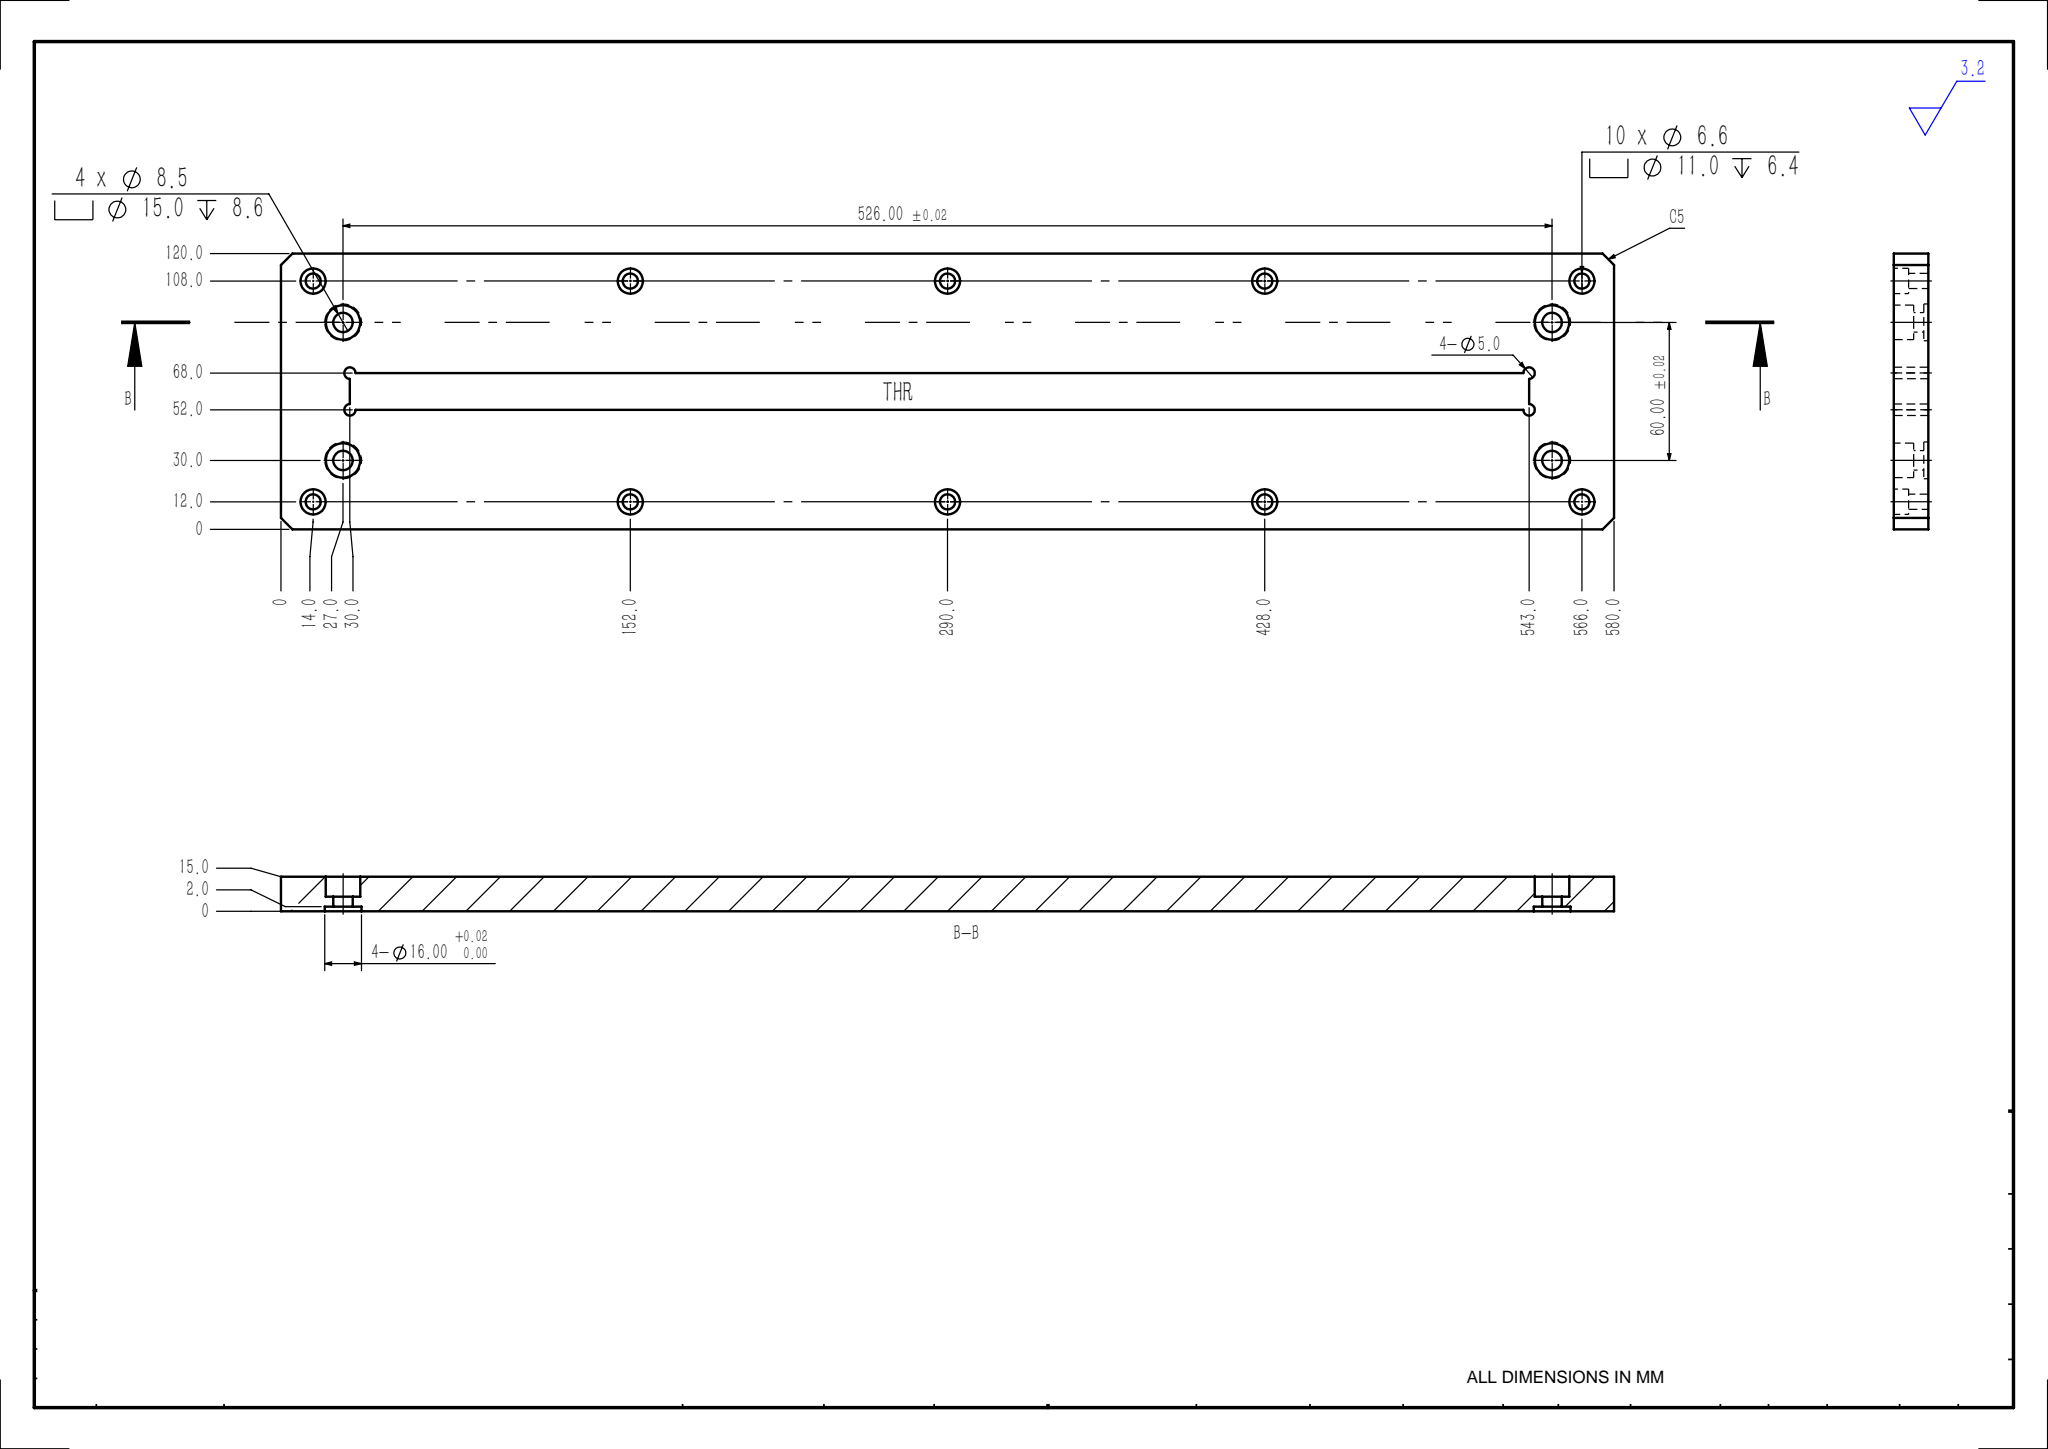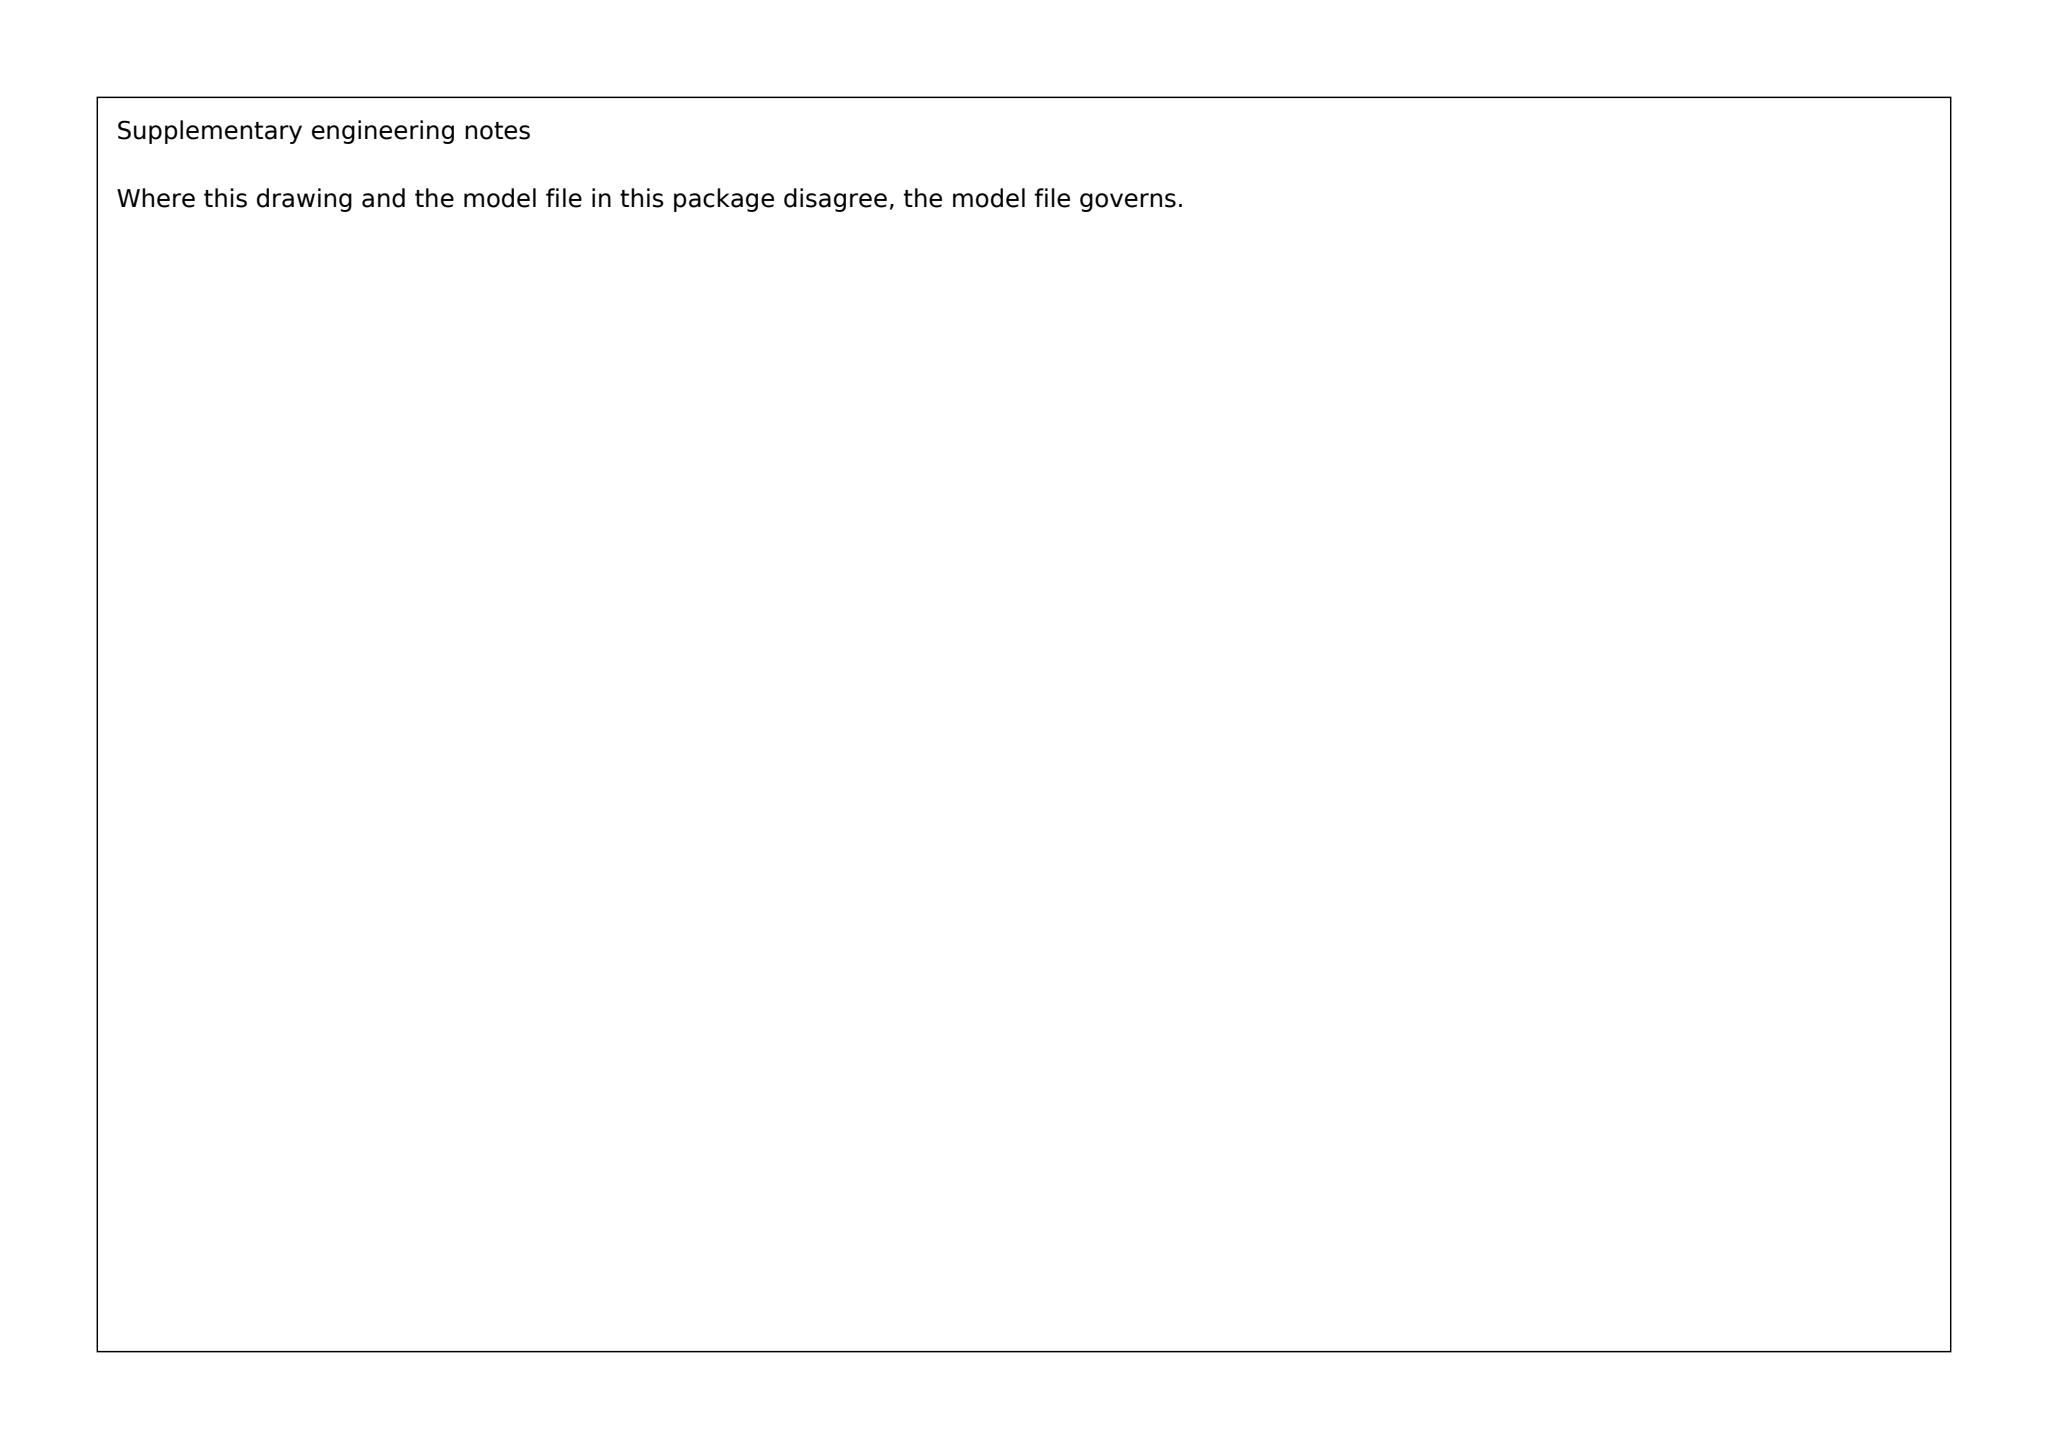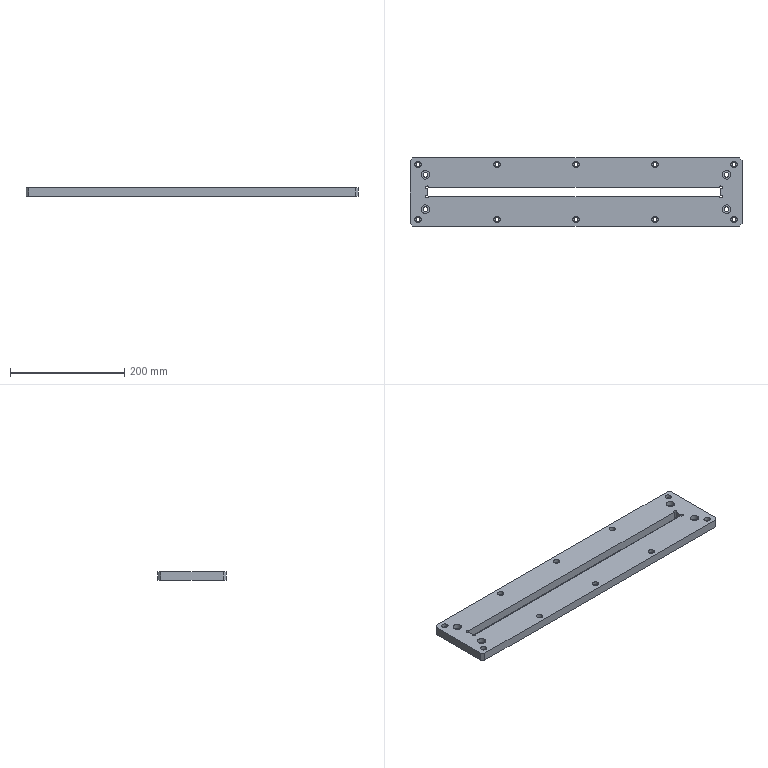Part | SolidWorks | mm | 1 solid | 102 faces | box 580 x 120 x 15 mm | volume 901536 mm3 | cylinder 70 | plane 32 | commonest cylinder face diameters 11 x20 6.6 x20 16 x8 15 x8 8.5 x8 5 x6
build123d program:
from build123d import *

# Parameters (mm, degrees)
SKETCH1_W                                       = 580
SKETCH1_H                                       = 120
BOSS_EXTRUDE1_DEPTH                             = 15
M8_HEX_SOCKET_HEAD_CAP_SCREW_CBORE1_D           = 8.5
M8_HEX_SOCKET_HEAD_CAP_SCREW_CBORE1_CBORE_D     = 15
M8_HEX_SOCKET_HEAD_CAP_SCREW_CBORE1_CBORE_DEPTH = 8.6
SKETCH5_R                                       = 8
CUT_EXTRUDE1_DEPTH                              = 2
CHAMFER1_SIZE                                   = 5
SKETCH6_W                                       = 513
SKETCH6_H                                       = 16
CUT_EXTRUDE2_DEPTH                              = 297.522
SKETCH7_R                                       = 2.5
CUT_EXTRUDE3_DEPTH                              = 297.522
M6_HEX_SOCKET_HEAD_CAP_SCREW_CBORE1_D           = 6.6
M6_HEX_SOCKET_HEAD_CAP_SCREW_CBORE1_CBORE_D     = 11
M6_HEX_SOCKET_HEAD_CAP_SCREW_CBORE1_CBORE_DEPTH = 6.4
LPATTERN1_COUNT                                 = 3
LPATTERN1_PITCH                                 = 138
LPATTERN1_COL_COUNT                             = 3
LPATTERN1_COL_PITCH                             = 138


with BuildPart() as part:
    # Sketch1 → Boss-Extrude1 (new body)
    with BuildSketch(Plane.XY):
        Rectangle(SKETCH1_W, SKETCH1_H)
    extrude(amount=BOSS_EXTRUDE1_DEPTH)

    # M8 Hex Socket Head Cap Screw CBORE1 (through all)
    with Locations(Plane.XY.offset(15)):
        with Locations((-263, 30), (-263, -30), (263, -30), (263, 30)):
            CounterBoreHole(M8_HEX_SOCKET_HEAD_CAP_SCREW_CBORE1_D / 2, M8_HEX_SOCKET_HEAD_CAP_SCREW_CBORE1_CBORE_D / 2, M8_HEX_SOCKET_HEAD_CAP_SCREW_CBORE1_CBORE_DEPTH)

    # Sketch5 → Cut-Extrude1 (cut)
    with BuildSketch(Plane(origin=(0, 0, 0), x_dir=(-1, 0, 0), z_dir=(0, 0, -1))):
        with Locations((-263, 30)):
            Circle(SKETCH5_R)
        with Locations((-263, -30)):
            Circle(SKETCH5_R)
        with Locations((263, -30)):
            Circle(SKETCH5_R)
        with Locations((263, 30)):
            Circle(SKETCH5_R)
    extrude(amount=-CUT_EXTRUDE1_DEPTH, mode=Mode.SUBTRACT)

    # Chamfer1
    chamfer1_edges = [part.edges().sort_by_distance(p)[0] for p in [
        (290, -60, 7.5),
        (-290, -60, 7.5),
        (-290, 60, 7.5),
        (290, 60, 7.5),
    ]]
    chamfer(chamfer1_edges, length=CHAMFER1_SIZE)

    # Sketch6 → Cut-Extrude2 (cut, through all)
    with BuildSketch(Plane.XY.offset(15)):
        with Locations((-3.5, 0)):
            Rectangle(SKETCH6_W, SKETCH6_H)
    extrude(amount=-CUT_EXTRUDE2_DEPTH, mode=Mode.SUBTRACT)

    # Sketch7 → Cut-Extrude3 (cut, through all)
    with BuildSketch(Plane.XY.offset(15)):
        with Locations((-260, -8)):
            Circle(SKETCH7_R)
        with Locations((-260, 8)):
            Circle(SKETCH7_R)
        with Locations((253, -8)):
            Circle(SKETCH7_R)
        with Locations((253, 8)):
            Circle(SKETCH7_R)
    extrude(amount=-CUT_EXTRUDE3_DEPTH, mode=Mode.SUBTRACT)

    # M6 Hex Socket Head Cap Screw CBORE1 (through all)
    with Locations(Plane.XY.offset(15)):
        with Locations((0, -48), (0, 48)):
            m6_hex_socket_head_cap_screw_cbore1 = CounterBoreHole(M6_HEX_SOCKET_HEAD_CAP_SCREW_CBORE1_D / 2, M6_HEX_SOCKET_HEAD_CAP_SCREW_CBORE1_CBORE_D / 2, M6_HEX_SOCKET_HEAD_CAP_SCREW_CBORE1_CBORE_DEPTH)

    # LPattern1: M6 Hex Socket Head Cap Screw CBORE1 ×3
    with Locations(*[(i * LPATTERN1_PITCH, 0, 0) for i in range(1, LPATTERN1_COUNT)]):
        add(m6_hex_socket_head_cap_screw_cbore1, mode=Mode.SUBTRACT)

    # LPattern1 col: M6 Hex Socket Head Cap Screw CBORE1 ×3
    with Locations(*[(-i * LPATTERN1_COL_PITCH, 0, 0) for i in range(1, LPATTERN1_COL_COUNT)]):
        add(m6_hex_socket_head_cap_screw_cbore1, mode=Mode.SUBTRACT)


solid = part.part